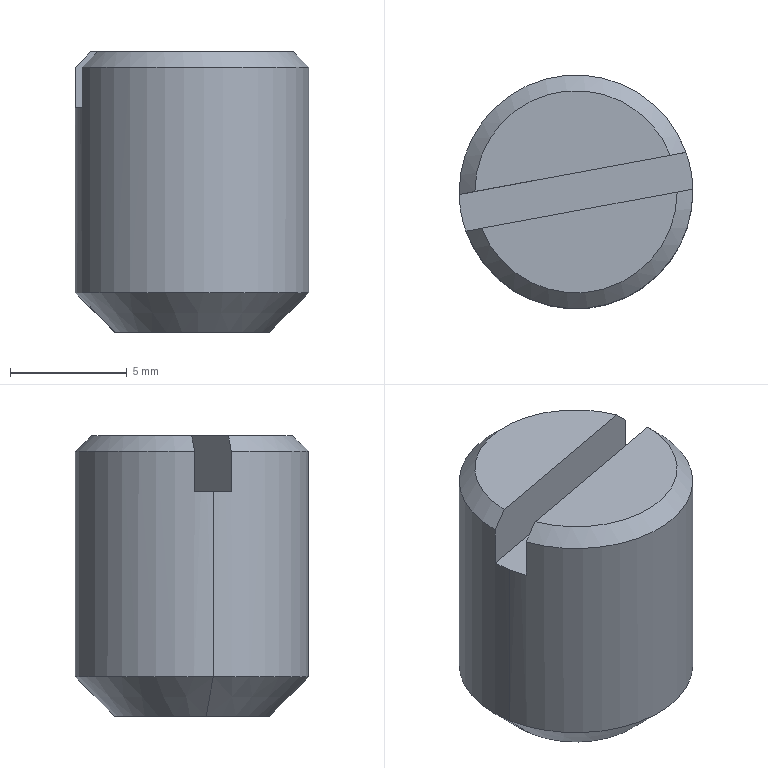Component | SolidWorks | GB73-85SlottedFlatPointSetScrewM10x12-1 | 1 solid | 12 faces | box 10 x 10 x 12 mm | volume 859 mm3 | plane 6 | cone 4 | cylinder 2 | commonest cylinder face diameters 10 x2 | material 14H Grade
build123d program:
from build123d import *

# Parameters (mm, degrees)
SKETCH3_W          = 2.4
SKETCH3_H          = 1.6
CUT_EXTRUDE1_DEPTH = 50


with BuildPart() as part:
    # Sketch2 → Base-Revolve (revolve)
    with BuildSketch(Plane.XY, mode=Mode.PRIVATE) as base_revolve_sk:
        Polygon((0, 0), (12, 0), (12, 3.32), (10.32, 5), (0.67, 5), (0, 4.33), align=None)
    revolve(base_revolve_sk.sketch.rotate(Axis((-0.5499, 0, 0), (1, 0, 0)), 90), axis=Axis((-0.5499, 0, 0), (1, 0, 0)))

    # Sketch3 → Cut-Extrude1 (cut, symmetric)
    with BuildSketch(Plane.XY):
        with Locations((1.2, 0)):
            Rectangle(SKETCH3_W, SKETCH3_H)
    extrude(amount=CUT_EXTRUDE1_DEPTH, both=True, mode=Mode.SUBTRACT)


solid = part.part

# Placed as in the assembly
solid = solid.moved(Location((-295, 84, 382), (90, -79.504, -90)))
STEP:
#1=CARTESIAN_POINT('',(-11.421,3.343,14.633));
#2=VERTEX_POINT('',#1);
#3=CARTESIAN_POINT('',(-11.808,3.271,14.633));
#4=VERTEX_POINT('',#3);
#5=CARTESIAN_POINT('',(-11.614,3.307,14.633));
#6=DIRECTION('',(0.,-0.,1.));
#7=DIRECTION('',(0.9833,0.1822,0.));
#8=AXIS2_PLACEMENT_3D('',#5,#6,#7);
#9=CIRCLE('',#8,0.1969);
#10=EDGE_CURVE('',#2,#4,#9,.T.);
#11=ORIENTED_EDGE('',*,*,#10,.T.);
#12=CARTESIAN_POINT('',(-11.808,3.271,14.945));
#13=VERTEX_POINT('',#12);
#14=CARTESIAN_POINT('',(-11.808,3.271,15.061));
#15=DIRECTION('',(0.,-0.,1.));
#16=VECTOR('',#15,39.37);
#17=LINE('',#14,#16);
#18=EDGE_CURVE('',#4,#13,#17,.T.);
#19=ORIENTED_EDGE('',*,*,#18,.T.);
#20=CARTESIAN_POINT('',(-11.811,3.303,14.945));
#21=VERTEX_POINT('',#20);
#22=CARTESIAN_POINT('',(-11.614,3.307,14.945));
#23=DIRECTION('',(-0.,0.,-1.));
#24=DIRECTION('',(-0.9833,-0.1822,0.));
#25=AXIS2_PLACEMENT_3D('',#22,#23,#24);
#26=CIRCLE('',#25,0.1969);
#27=EDGE_CURVE('',#13,#21,#26,.T.);
#28=ORIENTED_EDGE('',*,*,#27,.T.);
#29=CARTESIAN_POINT('',(-11.811,3.303,15.013));
#30=VERTEX_POINT('',#29);
#31=CARTESIAN_POINT('',(-11.811,3.303,15.061));
#32=DIRECTION('',(0.,-0.,1.));
#33=VECTOR('',#32,39.37);
#34=LINE('',#31,#33);
#35=EDGE_CURVE('',#21,#30,#34,.T.);
#36=ORIENTED_EDGE('',*,*,#35,.T.);
#37=CARTESIAN_POINT('',(-11.429,3.373,15.013));
#38=VERTEX_POINT('',#37);
#39=CARTESIAN_POINT('',(-11.614,3.307,15.013));
#40=DIRECTION('',(0.,-0.,1.));
#41=DIRECTION('',(0.9833,0.1822,0.));
#42=AXIS2_PLACEMENT_3D('',#39,#40,#41);
#43=CIRCLE('',#42,0.1969);
#44=EDGE_CURVE('',#38,#30,#43,.T.);
#45=ORIENTED_EDGE('',*,*,#44,.F.);
#46=CARTESIAN_POINT('',(-11.429,3.373,14.945));
#47=VERTEX_POINT('',#46);
#48=CARTESIAN_POINT('',(-11.429,3.373,15.061));
#49=DIRECTION('',(-0.,0.,-1.));
#50=VECTOR('',#49,39.37);
#51=LINE('',#48,#50);
#52=EDGE_CURVE('',#38,#47,#51,.T.);
#53=ORIENTED_EDGE('',*,*,#52,.T.);
#54=CARTESIAN_POINT('',(-11.421,3.343,14.945));
#55=VERTEX_POINT('',#54);
#56=CARTESIAN_POINT('',(-11.614,3.307,14.945));
#57=DIRECTION('',(-0.,0.,-1.));
#58=DIRECTION('',(-0.9833,-0.1822,0.));
#59=AXIS2_PLACEMENT_3D('',#56,#57,#58);
#60=CIRCLE('',#59,0.1969);
#61=EDGE_CURVE('',#47,#55,#60,.T.);
#62=ORIENTED_EDGE('',*,*,#61,.T.);
#63=CARTESIAN_POINT('',(-11.421,3.343,15.061));
#64=DIRECTION('',(0.,-0.,1.));
#65=VECTOR('',#64,39.37);
#66=LINE('',#63,#65);
#67=EDGE_CURVE('',#2,#55,#66,.T.);
#68=ORIENTED_EDGE('',*,*,#67,.F.);
#69=EDGE_LOOP('',(#11,#19,#28,#36,#45,#53,#62,#68));
#70=FACE_OUTER_BOUND('',#69,.T.);
#71=CARTESIAN_POINT('',(-11.614,3.307,15.061));
#72=DIRECTION('',(0.,-0.,1.));
#73=DIRECTION('',(0.9833,0.1822,0.));
#74=AXIS2_PLACEMENT_3D('',#71,#72,#73);
#75=CYLINDRICAL_SURFACE('',#74,0.1969);
#76=ADVANCED_FACE('',(#70),#75,.T.);
#77=CARTESIAN_POINT('',(-11.486,3.331,14.567));
#78=VERTEX_POINT('',#77);
#79=CARTESIAN_POINT('',(-11.743,3.283,14.567));
#80=VERTEX_POINT('',#79);
#81=CARTESIAN_POINT('',(-11.614,3.307,14.567));
#82=DIRECTION('',(0.,-0.,1.));
#83=DIRECTION('',(0.9833,0.1822,0.));
#84=AXIS2_PLACEMENT_3D('',#81,#82,#83);
#85=CIRCLE('',#84,0.1307);
#86=EDGE_CURVE('',#78,#80,#85,.T.);
#87=ORIENTED_EDGE('',*,*,#86,.T.);
#88=CARTESIAN_POINT('',(-11.743,3.283,14.567));
#89=DIRECTION('',(-0.6953,-0.1288,0.7071));
#90=VECTOR('',#89,39.37);
#91=LINE('',#88,#90);
#92=EDGE_CURVE('',#80,#4,#91,.T.);
#93=ORIENTED_EDGE('',*,*,#92,.T.);
#94=ORIENTED_EDGE('',*,*,#10,.F.);
#95=CARTESIAN_POINT('',(-11.486,3.331,14.567));
#96=DIRECTION('',(0.6953,0.1288,0.7071));
#97=VECTOR('',#96,39.37);
#98=LINE('',#95,#97);
#99=EDGE_CURVE('',#78,#2,#98,.T.);
#100=ORIENTED_EDGE('',*,*,#99,.F.);
#101=EDGE_LOOP('',(#87,#93,#94,#100));
#102=FACE_OUTER_BOUND('',#101,.T.);
#103=CARTESIAN_POINT('',(-11.614,3.307,14.567));
#104=DIRECTION('',(0.,-0.,1.));
#105=DIRECTION('',(0.9833,0.1822,0.));
#106=AXIS2_PLACEMENT_3D('',#103,#104,#105);
#107=CONICAL_SURFACE('',#106,0.1307,0.7854);
#108=ADVANCED_FACE('',(#102),#107,.T.);
#109=CARTESIAN_POINT('',(-11.455,3.369,15.039));
#110=VERTEX_POINT('',#109);
#111=CARTESIAN_POINT('',(-11.785,3.308,15.039));
#112=VERTEX_POINT('',#111);
#113=CARTESIAN_POINT('',(-11.614,3.307,15.039));
#114=DIRECTION('',(0.,-0.,1.));
#115=DIRECTION('',(0.9833,0.1822,0.));
#116=AXIS2_PLACEMENT_3D('',#113,#114,#115);
#117=CIRCLE('',#116,0.1705);
#118=EDGE_CURVE('',#110,#112,#117,.T.);
#119=ORIENTED_EDGE('',*,*,#118,.T.);
#120=CARTESIAN_POINT('',(-13.555,2.979,15.039));
#121=DIRECTION('',(0.9833,0.1822,-0.));
#122=VECTOR('',#121,39.37);
#123=LINE('',#120,#122);
#124=EDGE_CURVE('',#112,#110,#123,.T.);
#125=ORIENTED_EDGE('',*,*,#124,.T.);
#126=EDGE_LOOP('',(#119,#125));
#127=FACE_OUTER_BOUND('',#126,.T.);
#128=CARTESIAN_POINT('',(-11.645,3.475,15.039));
#129=DIRECTION('',(-0.,0.,-1.));
#130=DIRECTION('',(-0.9833,-0.1822,0.));
#131=AXIS2_PLACEMENT_3D('',#128,#129,#130);
#132=PLANE('',#131);
#133=ADVANCED_FACE('',(#127),#132,.F.);
#134=ORIENTED_EDGE('',*,*,#44,.T.);
#135=CARTESIAN_POINT('',(-11.811,3.303,15.013));
#136=CARTESIAN_POINT('',(-11.802,3.304,15.022));
#137=CARTESIAN_POINT('',(-11.793,3.306,15.031));
#138=CARTESIAN_POINT('',(-11.785,3.308,15.039));
#139=B_SPLINE_CURVE_WITH_KNOTS('',3,(#135,#136,#137,#138),.UNSPECIFIED.,.F.,.F.,(4,4),(0.00853,0.009484),.UNSPECIFIED.);
#140=EDGE_CURVE('',#30,#112,#139,.T.);
#141=ORIENTED_EDGE('',*,*,#140,.T.);
#142=ORIENTED_EDGE('',*,*,#118,.F.);
#143=CARTESIAN_POINT('',(-11.455,3.369,15.039));
#144=CARTESIAN_POINT('',(-11.446,3.37,15.031));
#145=CARTESIAN_POINT('',(-11.438,3.372,15.022));
#146=CARTESIAN_POINT('',(-11.429,3.373,15.013));
#147=B_SPLINE_CURVE_WITH_KNOTS('',3,(#143,#144,#145,#146),.UNSPECIFIED.,.F.,.F.,(4,4),(0.0207,0.02166),.UNSPECIFIED.);
#148=EDGE_CURVE('',#110,#38,#147,.T.);
#149=ORIENTED_EDGE('',*,*,#148,.T.);
#150=EDGE_LOOP('',(#134,#141,#142,#149));
#151=FACE_OUTER_BOUND('',#150,.T.);
#152=CARTESIAN_POINT('',(-11.614,3.307,15.013));
#153=DIRECTION('',(-0.,0.,-1.));
#154=DIRECTION('',(-0.9833,-0.1822,0.));
#155=AXIS2_PLACEMENT_3D('',#152,#153,#154);
#156=CONICAL_SURFACE('',#155,0.1969,0.7854);
#157=ADVANCED_FACE('',(#151),#156,.T.);
#158=CARTESIAN_POINT('',(-11.773,3.246,15.039));
#159=VERTEX_POINT('',#158);
#160=CARTESIAN_POINT('',(-11.444,3.307,15.039));
#161=VERTEX_POINT('',#160);
#162=CARTESIAN_POINT('',(-11.614,3.307,15.039));
#163=DIRECTION('',(0.,-0.,1.));
#164=DIRECTION('',(0.9833,0.1822,0.));
#165=AXIS2_PLACEMENT_3D('',#162,#163,#164);
#166=CIRCLE('',#165,0.1705);
#167=EDGE_CURVE('',#159,#161,#166,.T.);
#168=ORIENTED_EDGE('',*,*,#167,.T.);
#169=CARTESIAN_POINT('',(-13.544,2.918,15.039));
#170=DIRECTION('',(0.9833,0.1822,-0.));
#171=VECTOR('',#170,39.37);
#172=LINE('',#169,#171);
#173=EDGE_CURVE('',#159,#161,#172,.T.);
#174=ORIENTED_EDGE('',*,*,#173,.F.);
#175=EDGE_LOOP('',(#168,#174));
#176=FACE_OUTER_BOUND('',#175,.T.);
#177=CARTESIAN_POINT('',(-11.645,3.475,15.039));
#178=DIRECTION('',(-0.,0.,-1.));
#179=DIRECTION('',(-0.9833,-0.1822,0.));
#180=AXIS2_PLACEMENT_3D('',#177,#178,#179);
#181=PLANE('',#180);
#182=ADVANCED_FACE('',(#176),#181,.F.);
#183=ORIENTED_EDGE('',*,*,#86,.F.);
#184=CARTESIAN_POINT('',(-11.614,3.307,14.567));
#185=DIRECTION('',(0.,-0.,1.));
#186=DIRECTION('',(0.9833,0.1822,0.));
#187=AXIS2_PLACEMENT_3D('',#184,#185,#186);
#188=CIRCLE('',#187,0.1307);
#189=EDGE_CURVE('',#80,#78,#188,.T.);
#190=ORIENTED_EDGE('',*,*,#189,.F.);
#191=EDGE_LOOP('',(#183,#190));
#192=FACE_OUTER_BOUND('',#191,.T.);
#193=CARTESIAN_POINT('',(-11.614,3.307,14.567));
#194=DIRECTION('',(0.,-0.,1.));
#195=DIRECTION('',(0.9833,0.1822,-0.));
#196=AXIS2_PLACEMENT_3D('',#193,#194,#195);
#197=PLANE('',#196);
#198=ADVANCED_FACE('',(#192),#197,.F.);
#199=ORIENTED_EDGE('',*,*,#92,.F.);
#200=ORIENTED_EDGE('',*,*,#189,.T.);
#201=ORIENTED_EDGE('',*,*,#99,.T.);
#202=CARTESIAN_POINT('',(-11.614,3.307,14.633));
#203=DIRECTION('',(0.,-0.,1.));
#204=DIRECTION('',(0.9833,0.1822,0.));
#205=AXIS2_PLACEMENT_3D('',#202,#203,#204);
#206=CIRCLE('',#205,0.1969);
#207=EDGE_CURVE('',#4,#2,#206,.T.);
#208=ORIENTED_EDGE('',*,*,#207,.F.);
#209=EDGE_LOOP('',(#199,#200,#201,#208));
#210=FACE_OUTER_BOUND('',#209,.T.);
#211=CARTESIAN_POINT('',(-11.614,3.307,14.567));
#212=DIRECTION('',(0.,-0.,1.));
#213=DIRECTION('',(0.9833,0.1822,0.));
#214=AXIS2_PLACEMENT_3D('',#211,#212,#213);
#215=CONICAL_SURFACE('',#214,0.1307,0.7854);
#216=ADVANCED_FACE('',(#210),#215,.T.);
#217=ORIENTED_EDGE('',*,*,#18,.F.);
#218=ORIENTED_EDGE('',*,*,#207,.T.);
#219=ORIENTED_EDGE('',*,*,#67,.T.);
#220=CARTESIAN_POINT('',(-11.417,3.312,14.945));
#221=VERTEX_POINT('',#220);
#222=CARTESIAN_POINT('',(-11.614,3.307,14.945));
#223=DIRECTION('',(-0.,0.,-1.));
#224=DIRECTION('',(-0.9833,-0.1822,0.));
#225=AXIS2_PLACEMENT_3D('',#222,#223,#224);
#226=CIRCLE('',#225,0.1969);
#227=EDGE_CURVE('',#55,#221,#226,.T.);
#228=ORIENTED_EDGE('',*,*,#227,.T.);
#229=CARTESIAN_POINT('',(-11.417,3.312,15.013));
#230=VERTEX_POINT('',#229);
#231=CARTESIAN_POINT('',(-11.417,3.312,15.061));
#232=DIRECTION('',(0.,-0.,1.));
#233=VECTOR('',#232,39.37);
#234=LINE('',#231,#233);
#235=EDGE_CURVE('',#221,#230,#234,.T.);
#236=ORIENTED_EDGE('',*,*,#235,.T.);
#237=CARTESIAN_POINT('',(-11.799,3.241,15.013));
#238=VERTEX_POINT('',#237);
#239=CARTESIAN_POINT('',(-11.614,3.307,15.013));
#240=DIRECTION('',(0.,-0.,1.));
#241=DIRECTION('',(0.9833,0.1822,0.));
#242=AXIS2_PLACEMENT_3D('',#239,#240,#241);
#243=CIRCLE('',#242,0.1969);
#244=EDGE_CURVE('',#238,#230,#243,.T.);
#245=ORIENTED_EDGE('',*,*,#244,.F.);
#246=CARTESIAN_POINT('',(-11.799,3.241,14.945));
#247=VERTEX_POINT('',#246);
#248=CARTESIAN_POINT('',(-11.799,3.241,15.061));
#249=DIRECTION('',(-0.,0.,-1.));
#250=VECTOR('',#249,39.37);
#251=LINE('',#248,#250);
#252=EDGE_CURVE('',#238,#247,#251,.T.);
#253=ORIENTED_EDGE('',*,*,#252,.T.);
#254=CARTESIAN_POINT('',(-11.614,3.307,14.945));
#255=DIRECTION('',(-0.,0.,-1.));
#256=DIRECTION('',(-0.9833,-0.1822,0.));
#257=AXIS2_PLACEMENT_3D('',#254,#255,#256);
#258=CIRCLE('',#257,0.1969);
#259=EDGE_CURVE('',#247,#13,#258,.T.);
#260=ORIENTED_EDGE('',*,*,#259,.T.);
#261=EDGE_LOOP('',(#217,#218,#219,#228,#236,#245,#253,#260));
#262=FACE_OUTER_BOUND('',#261,.T.);
#263=CARTESIAN_POINT('',(-11.614,3.307,15.061));
#264=DIRECTION('',(0.,-0.,1.));
#265=DIRECTION('',(0.9833,0.1822,0.));
#266=AXIS2_PLACEMENT_3D('',#263,#264,#265);
#267=CYLINDRICAL_SURFACE('',#266,0.1969);
#268=ADVANCED_FACE('',(#262),#267,.T.);
#269=ORIENTED_EDGE('',*,*,#244,.T.);
#270=CARTESIAN_POINT('',(-11.417,3.312,15.013));
#271=CARTESIAN_POINT('',(-11.426,3.31,15.022));
#272=CARTESIAN_POINT('',(-11.435,3.308,15.031));
#273=CARTESIAN_POINT('',(-11.444,3.307,15.039));
#274=B_SPLINE_CURVE_WITH_KNOTS('',3,(#270,#271,#272,#273),.UNSPECIFIED.,.F.,.F.,(4,4),(0.00853,0.009484),.UNSPECIFIED.);
#275=EDGE_CURVE('',#230,#161,#274,.T.);
#276=ORIENTED_EDGE('',*,*,#275,.T.);
#277=ORIENTED_EDGE('',*,*,#167,.F.);
#278=CARTESIAN_POINT('',(-11.773,3.246,15.039));
#279=CARTESIAN_POINT('',(-11.782,3.244,15.031));
#280=CARTESIAN_POINT('',(-11.791,3.242,15.022));
#281=CARTESIAN_POINT('',(-11.799,3.241,15.013));
#282=B_SPLINE_CURVE_WITH_KNOTS('',3,(#278,#279,#280,#281),.UNSPECIFIED.,.F.,.F.,(4,4),(0.0207,0.02166),.UNSPECIFIED.);
#283=EDGE_CURVE('',#159,#238,#282,.T.);
#284=ORIENTED_EDGE('',*,*,#283,.T.);
#285=EDGE_LOOP('',(#269,#276,#277,#284));
#286=FACE_OUTER_BOUND('',#285,.T.);
#287=CARTESIAN_POINT('',(-11.614,3.307,15.013));
#288=DIRECTION('',(-0.,0.,-1.));
#289=DIRECTION('',(-0.9833,-0.1822,0.));
#290=AXIS2_PLACEMENT_3D('',#287,#288,#289);
#291=CONICAL_SURFACE('',#290,0.1969,0.7854);
#292=ADVANCED_FACE('',(#286),#291,.T.);
#293=CARTESIAN_POINT('',(-13.555,2.979,14.945));
#294=DIRECTION('',(0.9833,0.1822,-0.));
#295=VECTOR('',#294,39.37);
#296=LINE('',#293,#295);
#297=EDGE_CURVE('',#21,#47,#296,.T.);
#298=ORIENTED_EDGE('',*,*,#297,.F.);
#299=ORIENTED_EDGE('',*,*,#27,.F.);
#300=ORIENTED_EDGE('',*,*,#259,.F.);
#301=CARTESIAN_POINT('',(-13.544,2.918,14.945));
#302=DIRECTION('',(0.9833,0.1822,-0.));
#303=VECTOR('',#302,39.37);
#304=LINE('',#301,#303);
#305=EDGE_CURVE('',#247,#221,#304,.T.);
#306=ORIENTED_EDGE('',*,*,#305,.T.);
#307=ORIENTED_EDGE('',*,*,#227,.F.);
#308=ORIENTED_EDGE('',*,*,#61,.F.);
#309=EDGE_LOOP('',(#298,#299,#300,#306,#307,#308));
#310=FACE_OUTER_BOUND('',#309,.T.);
#311=CARTESIAN_POINT('',(-13.544,2.918,14.945));
#312=DIRECTION('',(-0.,0.,-1.));
#313=DIRECTION('',(-0.9833,-0.1822,0.));
#314=AXIS2_PLACEMENT_3D('',#311,#312,#313);
#315=PLANE('',#314);
#316=ADVANCED_FACE('',(#310),#315,.F.);
#317=ORIENTED_EDGE('',*,*,#297,.T.);
#318=ORIENTED_EDGE('',*,*,#52,.F.);
#319=ORIENTED_EDGE('',*,*,#148,.F.);
#320=ORIENTED_EDGE('',*,*,#124,.F.);
#321=ORIENTED_EDGE('',*,*,#140,.F.);
#322=ORIENTED_EDGE('',*,*,#35,.F.);
#323=EDGE_LOOP('',(#317,#318,#319,#320,#321,#322));
#324=FACE_OUTER_BOUND('',#323,.T.);
#325=CARTESIAN_POINT('',(-13.555,2.979,15.039));
#326=DIRECTION('',(-0.1822,0.9833,0.));
#327=DIRECTION('',(0.9833,0.1822,-0.));
#328=AXIS2_PLACEMENT_3D('',#325,#326,#327);
#329=PLANE('',#328);
#330=ADVANCED_FACE('',(#324),#329,.F.);
#331=ORIENTED_EDGE('',*,*,#305,.F.);
#332=ORIENTED_EDGE('',*,*,#252,.F.);
#333=ORIENTED_EDGE('',*,*,#283,.F.);
#334=ORIENTED_EDGE('',*,*,#173,.T.);
#335=ORIENTED_EDGE('',*,*,#275,.F.);
#336=ORIENTED_EDGE('',*,*,#235,.F.);
#337=EDGE_LOOP('',(#331,#332,#333,#334,#335,#336));
#338=FACE_OUTER_BOUND('',#337,.T.);
#339=CARTESIAN_POINT('',(-13.544,2.918,15.039));
#340=DIRECTION('',(0.1822,-0.9833,-0.));
#341=DIRECTION('',(-0.,0.,-1.));
#342=AXIS2_PLACEMENT_3D('',#339,#340,#341);
#343=PLANE('',#342);
#344=ADVANCED_FACE('',(#338),#343,.F.);
#345=CLOSED_SHELL('',(#76,#108,#133,#157,#182,#198,#216,#268,#292,#316,#330,#344));
#346=MANIFOLD_SOLID_BREP('',#345);
#347=CARTESIAN_POINT('',(0.,0.,0.));
#348=DIRECTION('',(0.,0.,1.));
#349=DIRECTION('',(1.,0.,0.));
#350=AXIS2_PLACEMENT_3D('',#347,#348,#349);
#351=(LENGTH_UNIT()NAMED_UNIT(*)SI_UNIT($,.METRE.));
#352=LENGTH_MEASURE_WITH_UNIT(LENGTH_MEASURE(0.0254),#351);
#353=DIMENSIONAL_EXPONENTS(1.,0.,0.,0.,0.,0.,0.);
#354=(CONVERSION_BASED_UNIT('',#352)LENGTH_UNIT()NAMED_UNIT(#353));
#355=UNCERTAINTY_MEASURE_WITH_UNIT(LENGTH_MEASURE(0.00001),#354,'','');
#356=(NAMED_UNIT(*)PLANE_ANGLE_UNIT()SI_UNIT($,.RADIAN.));
#357=(NAMED_UNIT(*)SI_UNIT($,.STERADIAN.)SOLID_ANGLE_UNIT());
#358=(GEOMETRIC_REPRESENTATION_CONTEXT(3)GLOBAL_UNCERTAINTY_ASSIGNED_CONTEXT((#355))GLOBAL_UNIT_ASSIGNED_CONTEXT((#354,#356,#357))REPRESENTATION_CONTEXT('',''));
#359=ADVANCED_BREP_SHAPE_REPRESENTATION('',(#346,#350),#358);
#360=COLOUR_RGB('',0.7922,0.8196,0.9333);
#361=FILL_AREA_STYLE_COLOUR('',#360);
#362=FILL_AREA_STYLE('',(#361));
#363=SURFACE_STYLE_FILL_AREA(#362);
#364=SURFACE_SIDE_STYLE('',(#363));
#365=SURFACE_STYLE_USAGE(.BOTH.,#364);
#366=PRESENTATION_STYLE_ASSIGNMENT((#365));
#367=STYLED_ITEM('',(#366),#346);
#368=(LENGTH_UNIT()NAMED_UNIT(*)SI_UNIT($,.METRE.));
#369=LENGTH_MEASURE_WITH_UNIT(LENGTH_MEASURE(0.0254),#368);
#370=DIMENSIONAL_EXPONENTS(1.,0.,0.,0.,0.,0.,0.);
#371=(CONVERSION_BASED_UNIT('',#369)LENGTH_UNIT()NAMED_UNIT(#370));
#372=UNCERTAINTY_MEASURE_WITH_UNIT(LENGTH_MEASURE(0.00001),#371,'','');
#373=(NAMED_UNIT(*)PLANE_ANGLE_UNIT()SI_UNIT($,.RADIAN.));
#374=(NAMED_UNIT(*)SI_UNIT($,.STERADIAN.)SOLID_ANGLE_UNIT());
#375=(GEOMETRIC_REPRESENTATION_CONTEXT(3)GLOBAL_UNCERTAINTY_ASSIGNED_CONTEXT((#372))GLOBAL_UNIT_ASSIGNED_CONTEXT((#371,#373,#374))REPRESENTATION_CONTEXT('',''));
#376=MECHANICAL_DESIGN_GEOMETRIC_PRESENTATION_REPRESENTATION('',(#367),#375);
#377=PRESENTATION_LAYER_ASSIGNMENT('','',(#367));